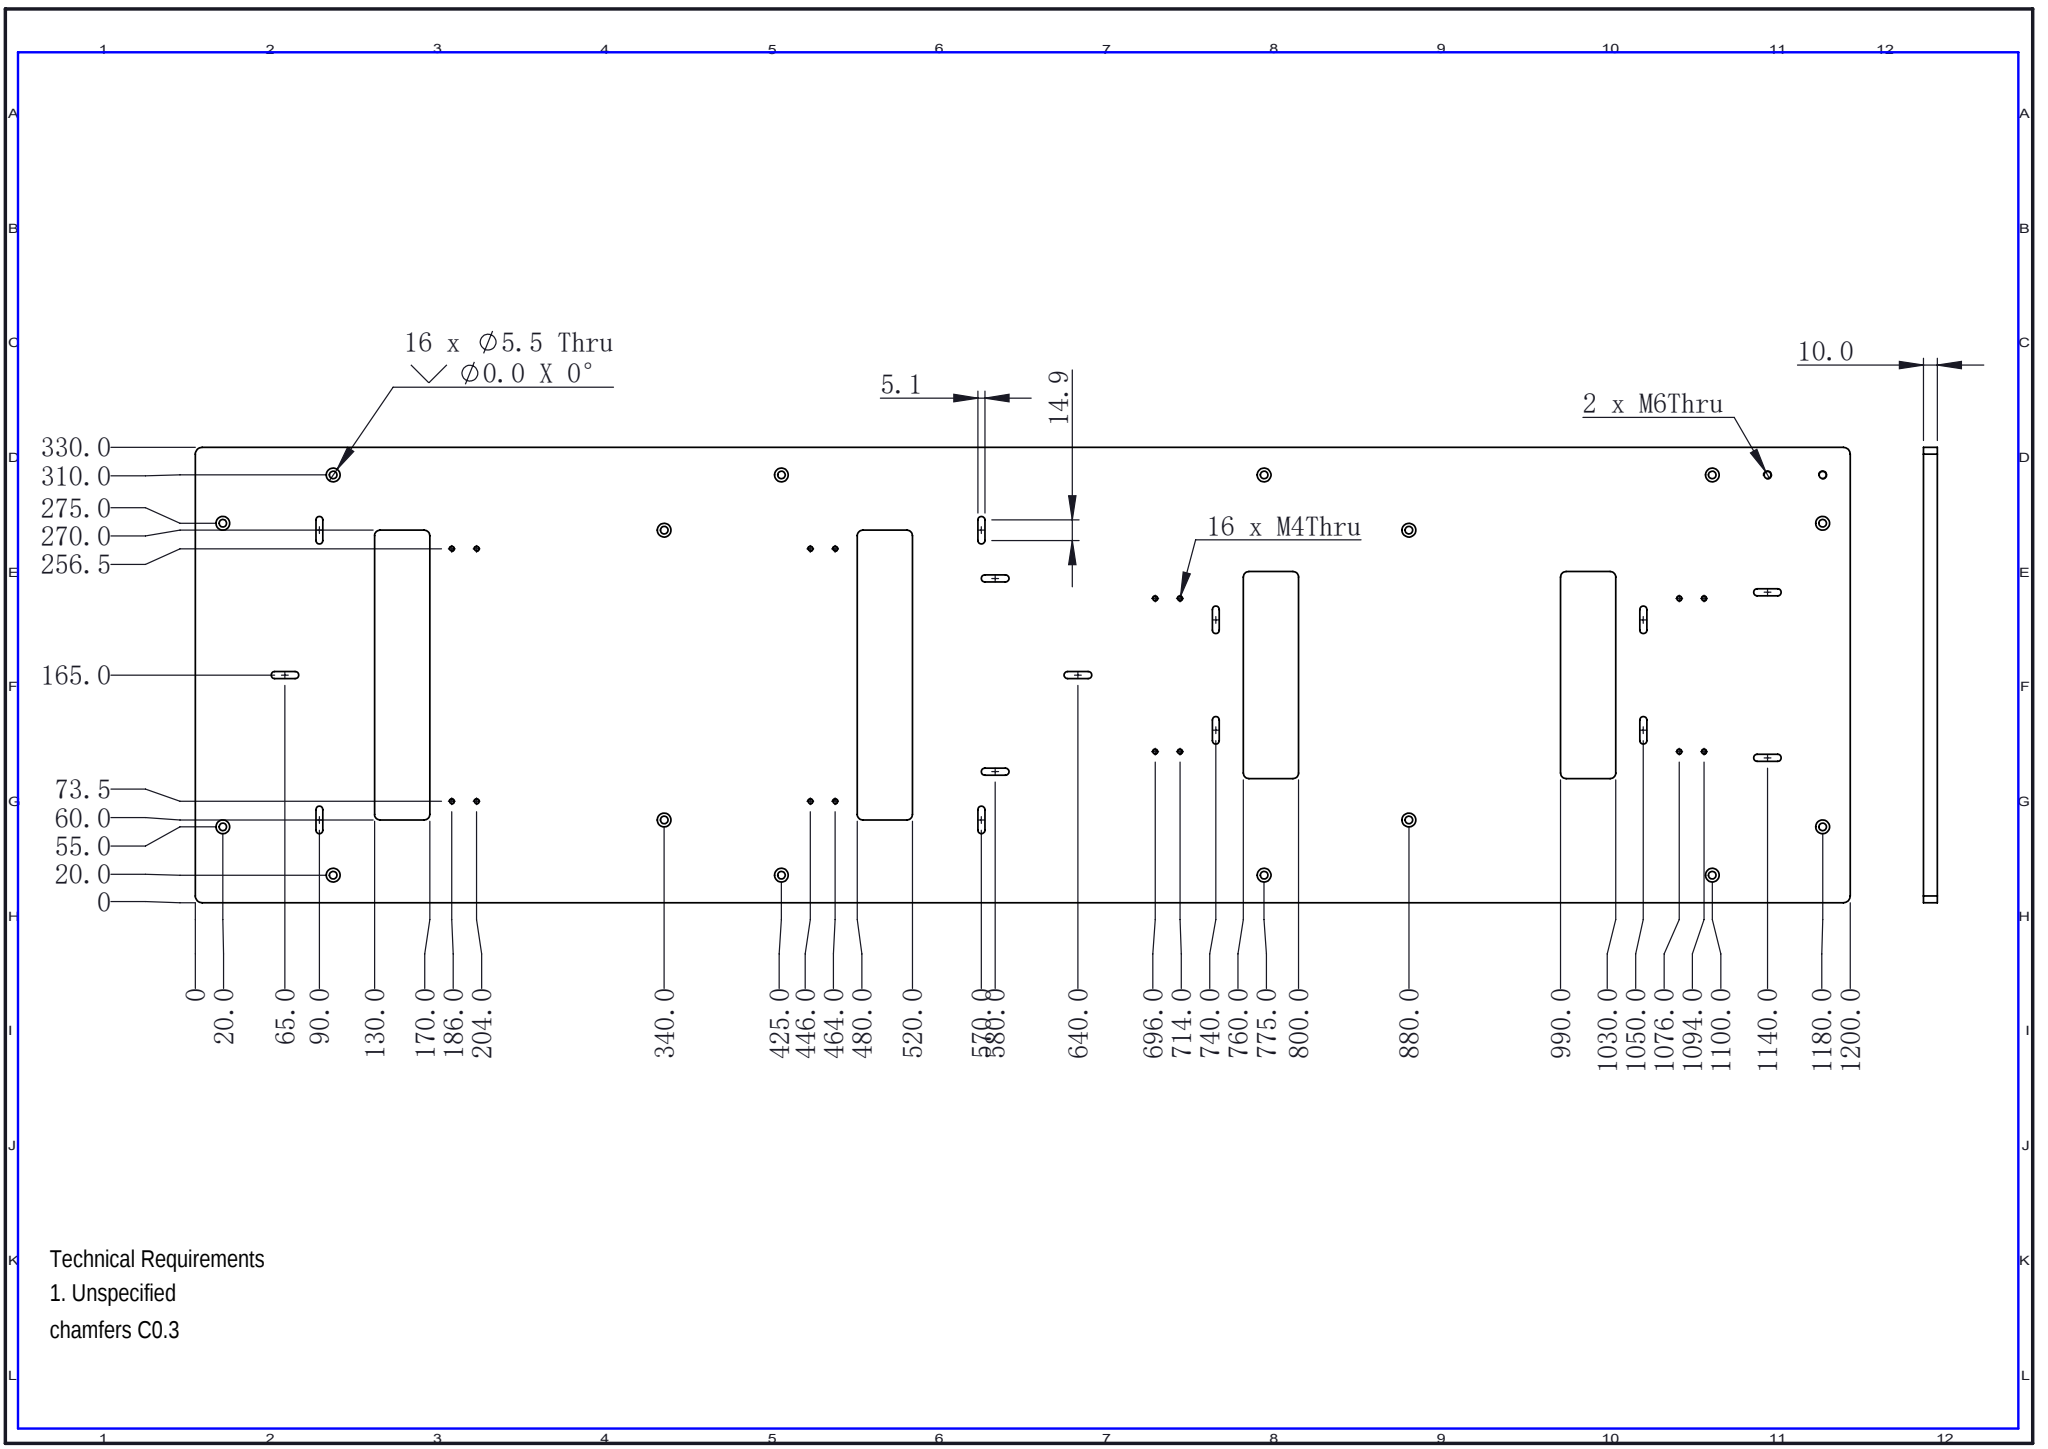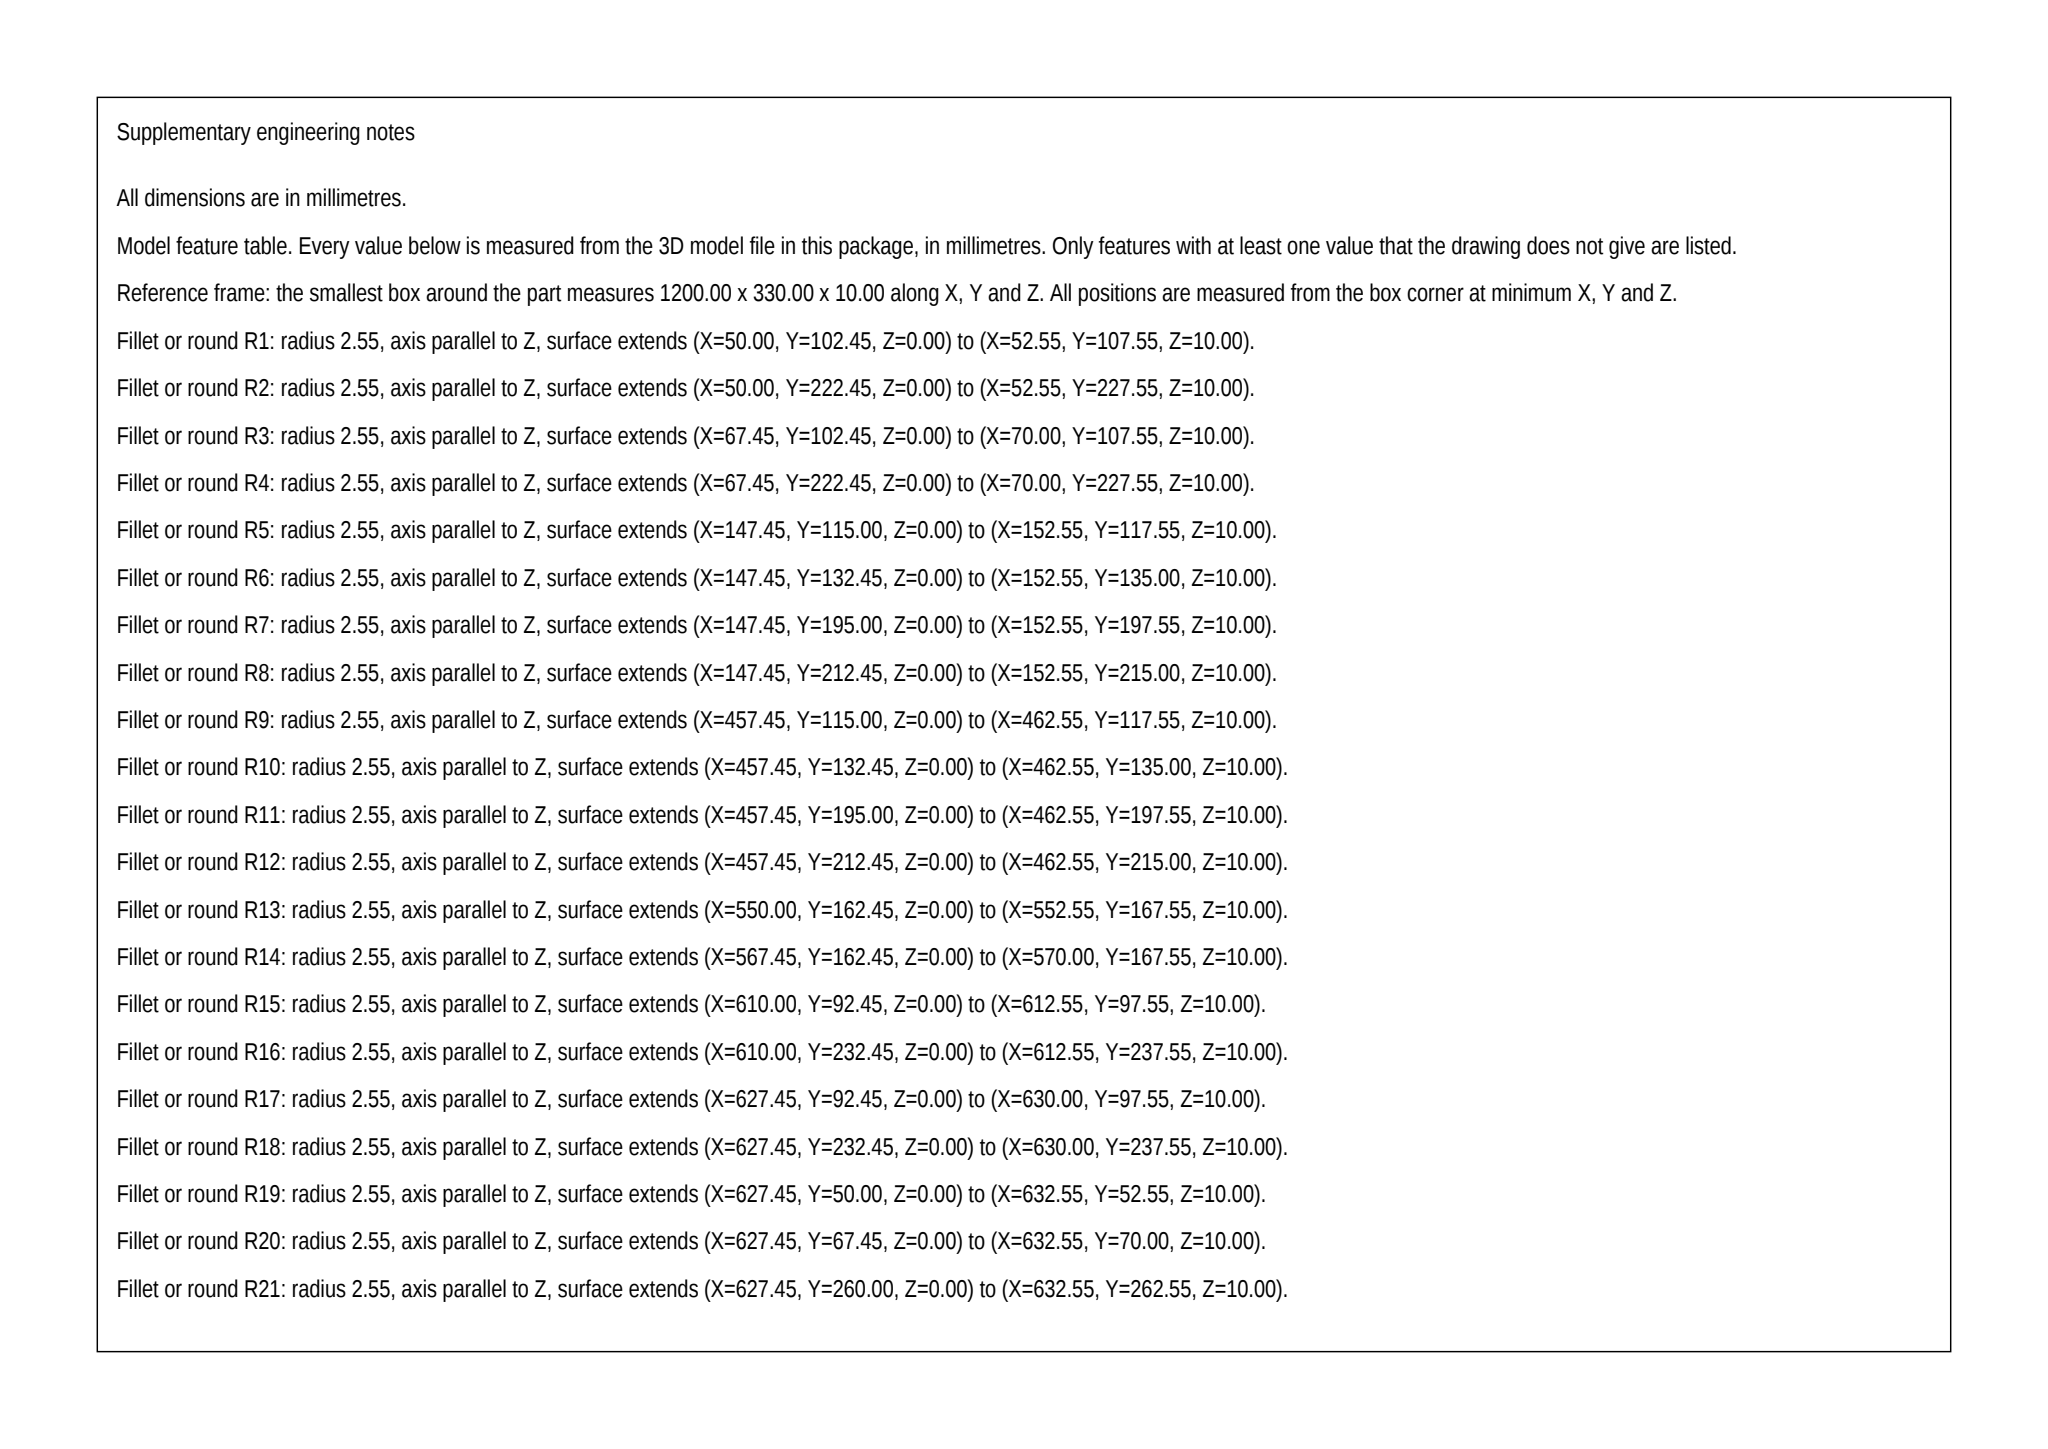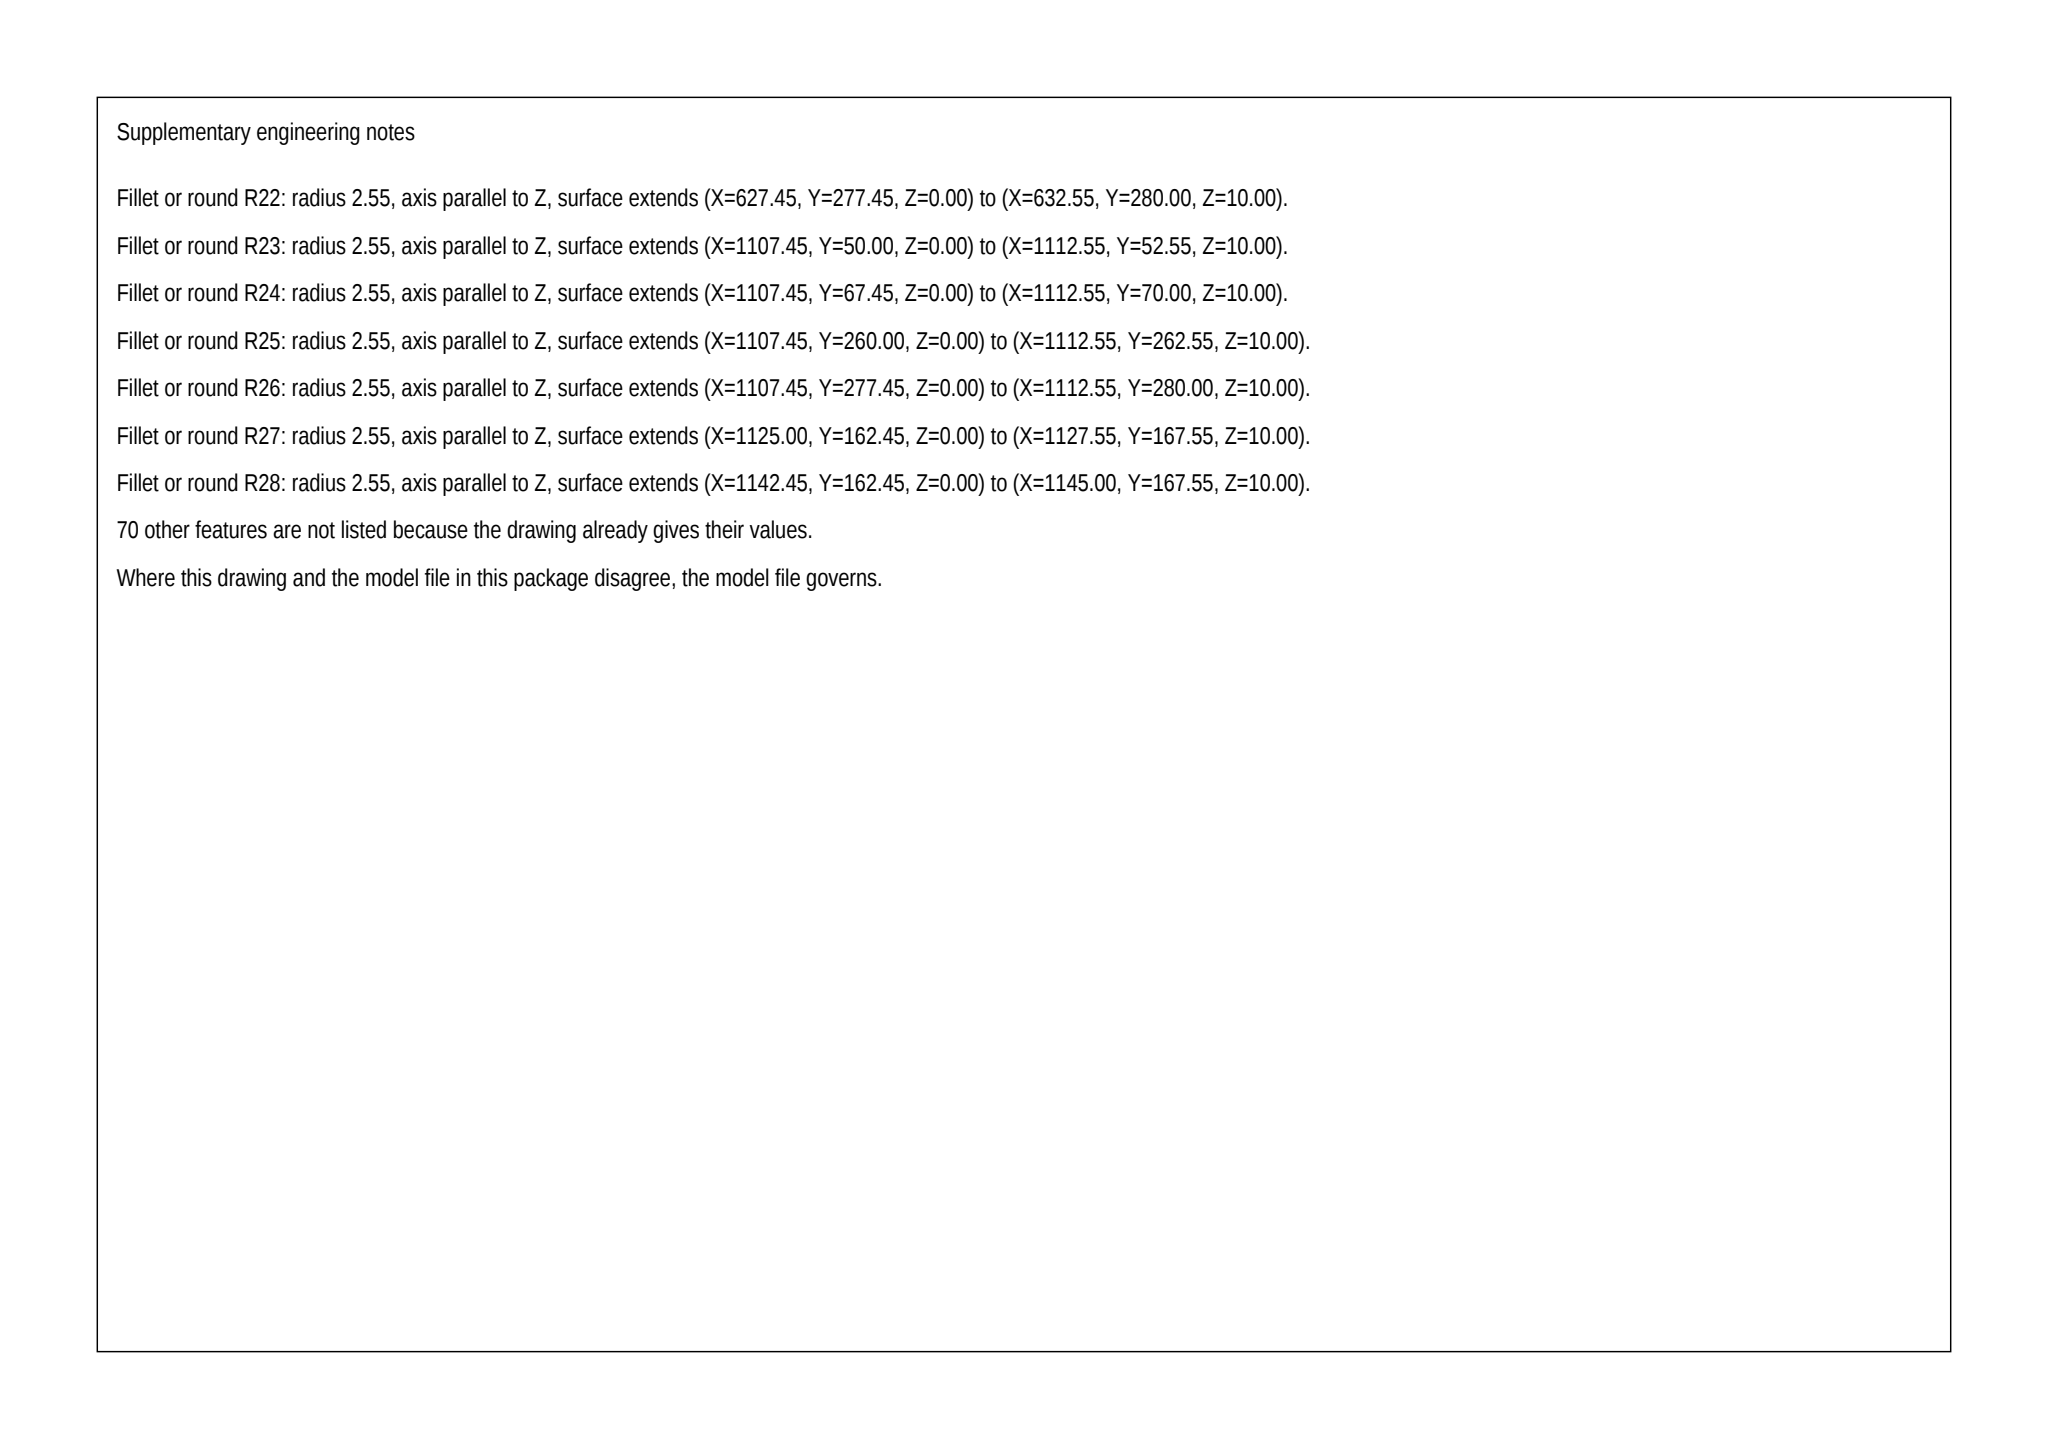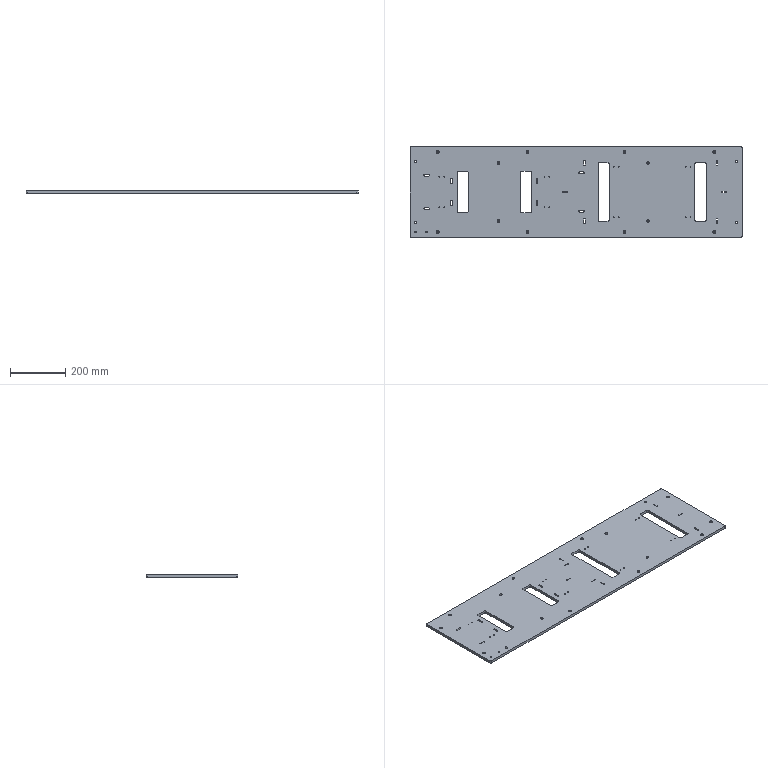Part | SolidWorks | mm | 1 solid | 220 faces | box 1200 x 330 x 10 mm | volume 3648541 mm3 | cylinder 154 | plane 66 | commonest cylinder face diameters 10 x36 5.1 x34 5.5 x32 3.3 x32 8 x16 5 x4